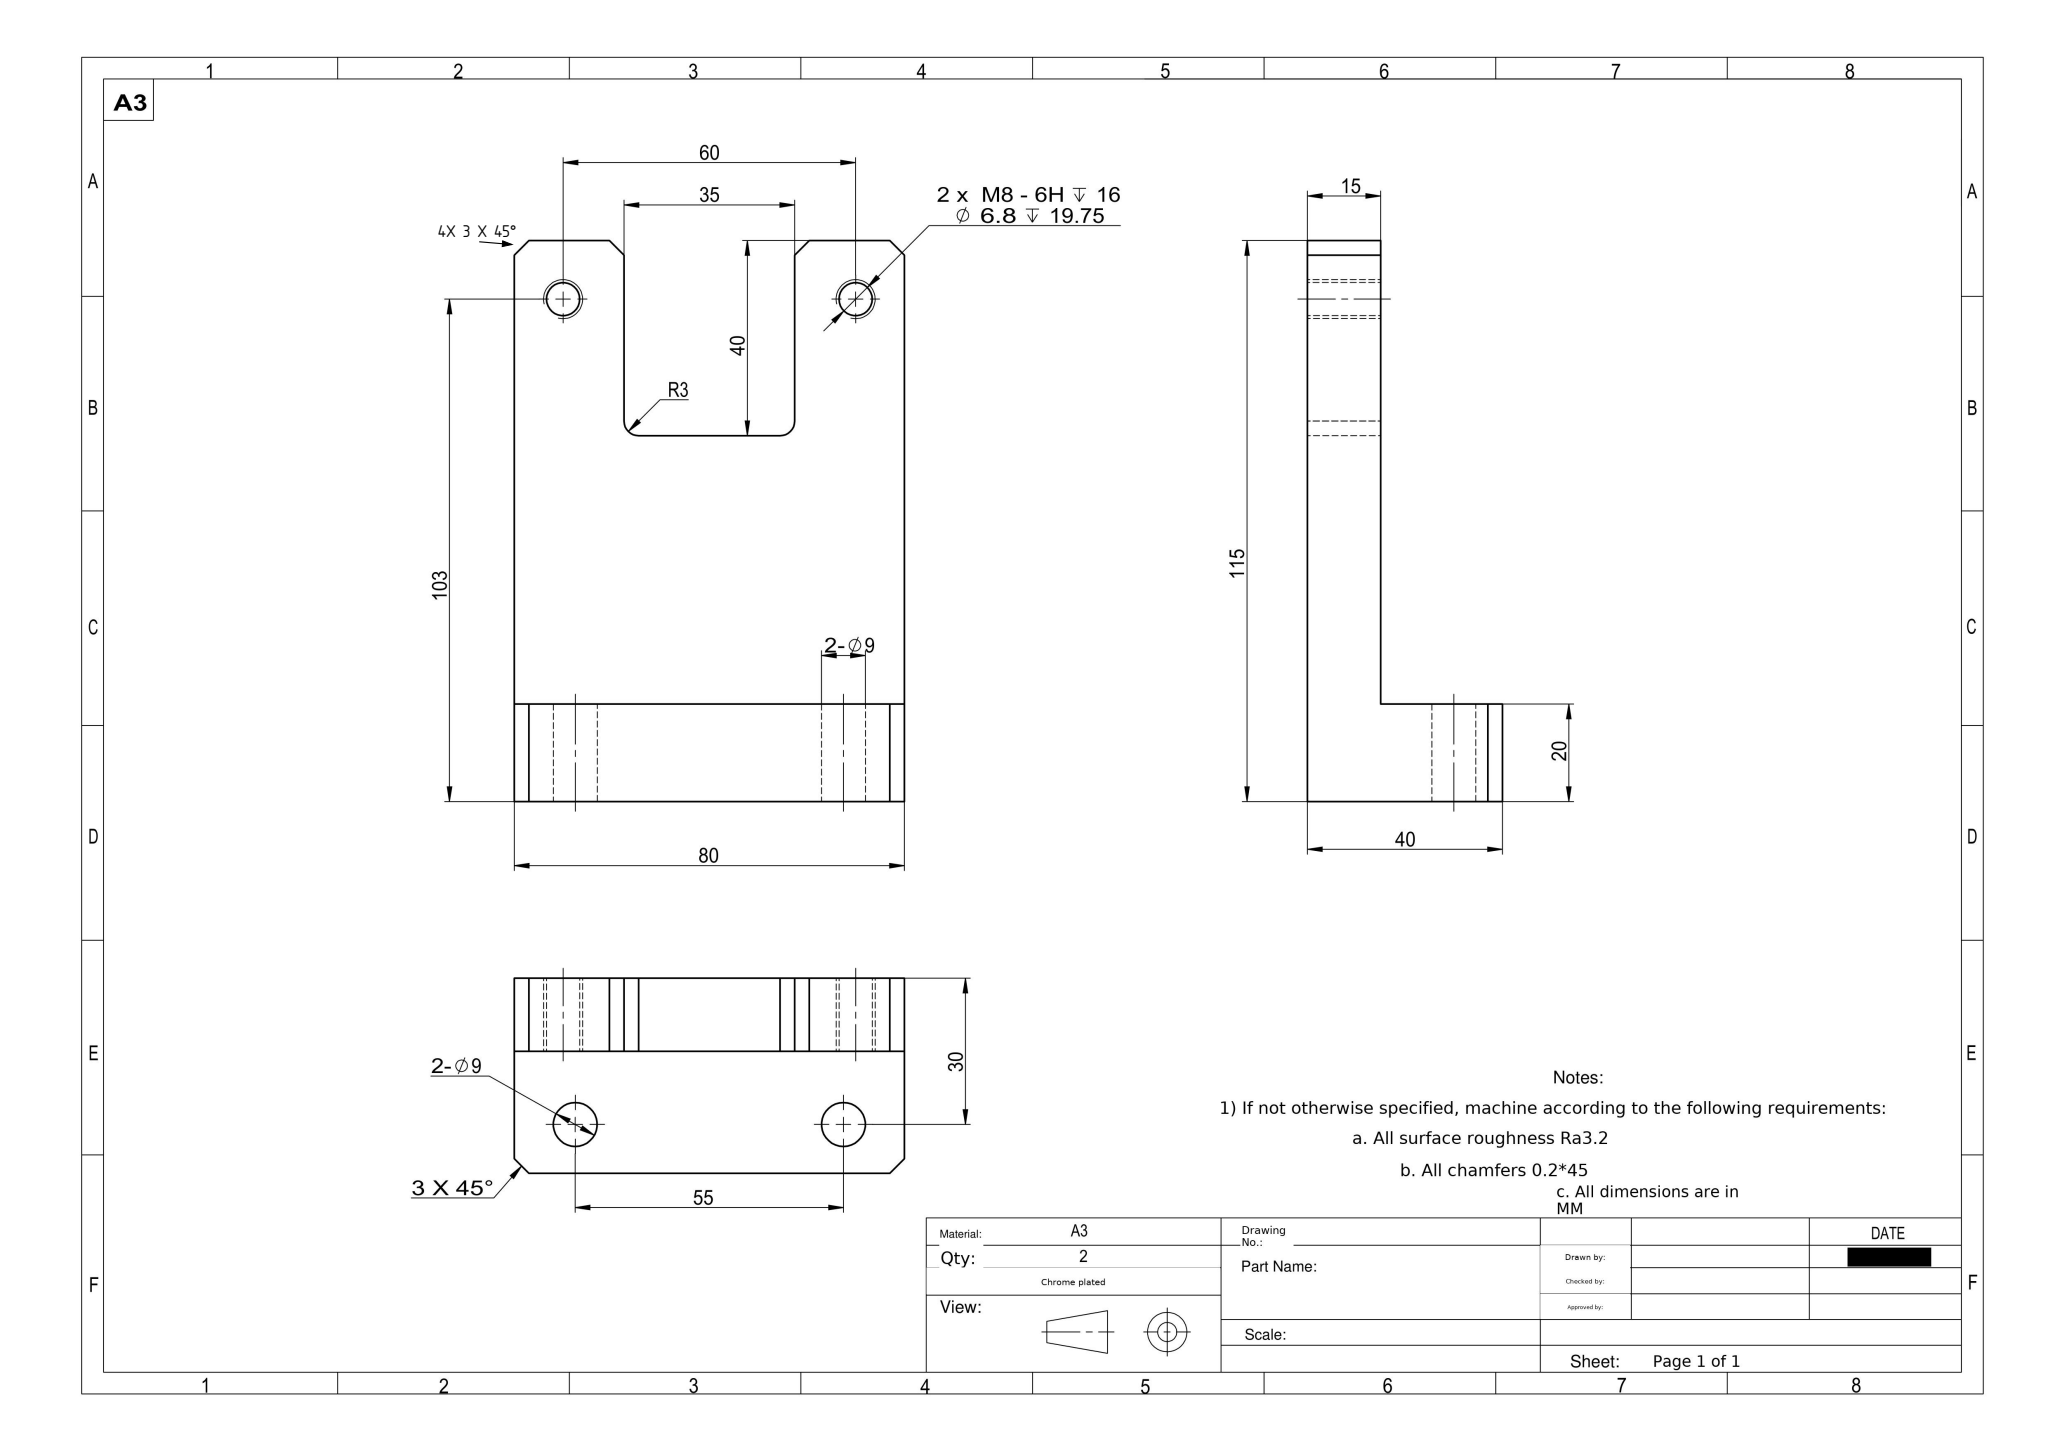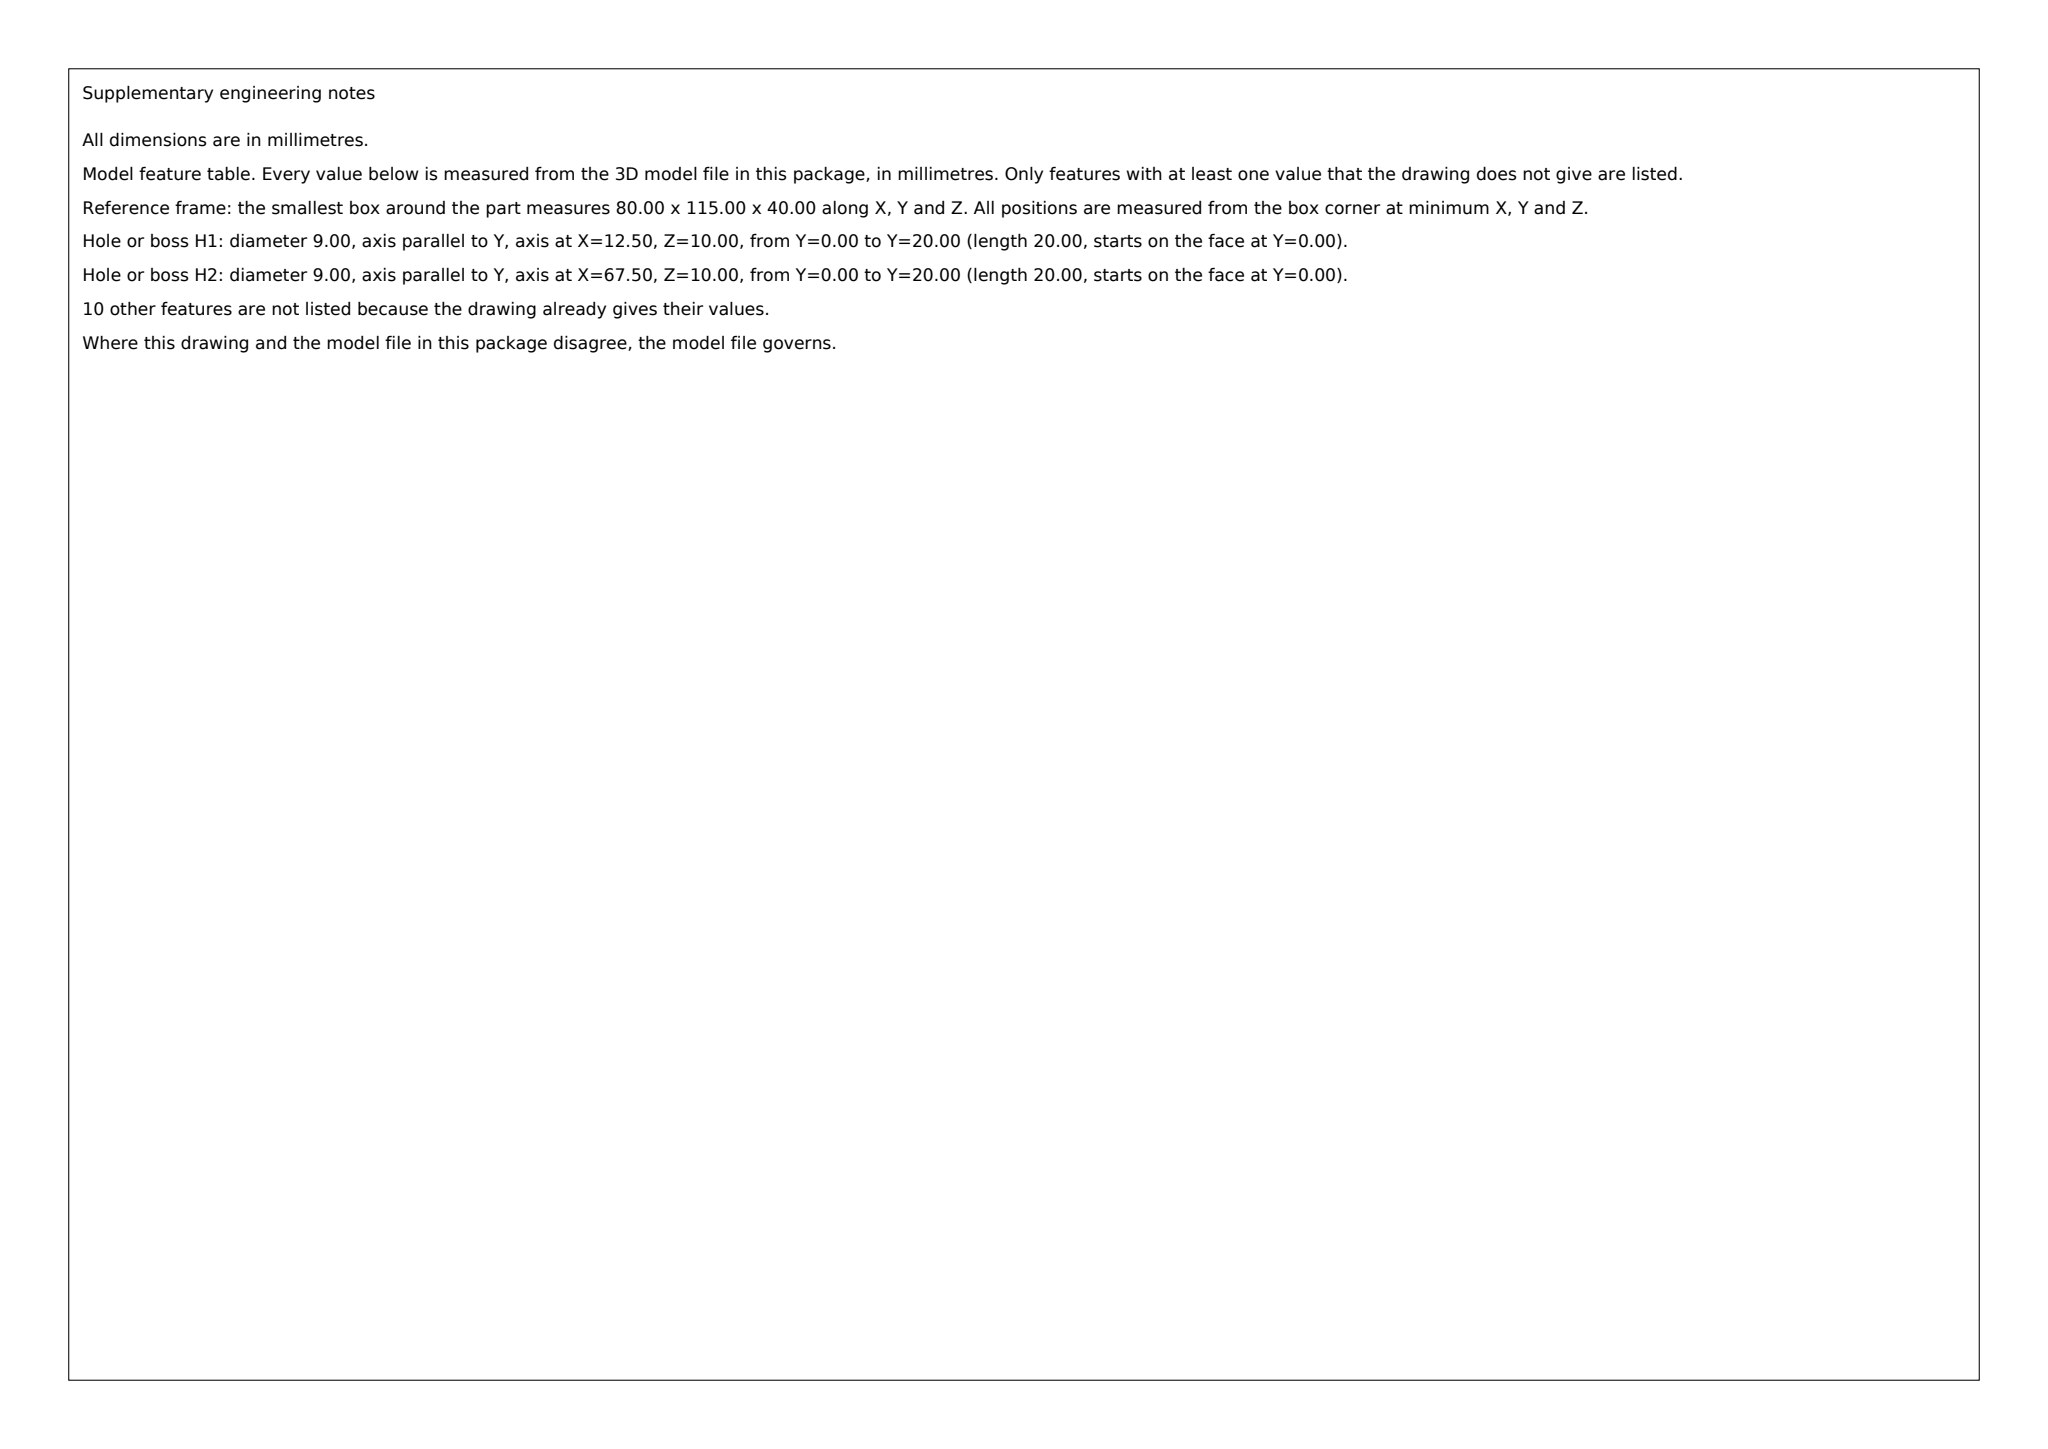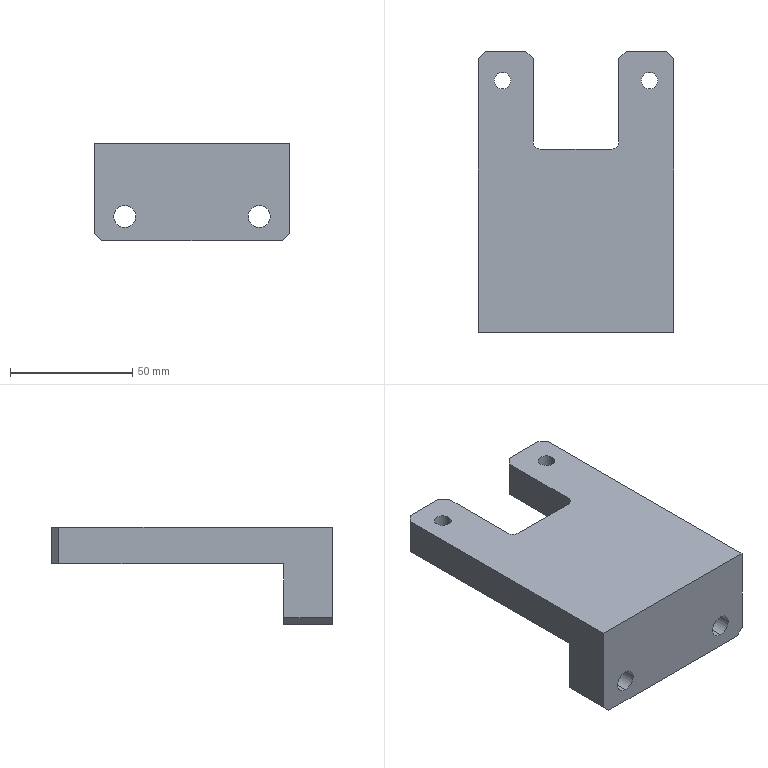Part | SolidWorks | mm | material A3 | 1 solid | 28 faces | box 80 x 115 x 40 mm | volume 152974 mm3 | plane 18 | cylinder 10 | commonest cylinder face diameters 6.8 x4 9 x4 6 x2
Drawing notes:
4X 3 X 45° CHAMFER ON TOP EDGE OF VERTICAL PLATE (15 THK), FULL THICKNESS; CHAMFER STARTS AT Y=112 FROM BOTTOM FACE, AT X=0, 19.5, 57.5 AND 77 FROM LEFT EDGE | from the solid: inclined_planes 4X angle_to_xyz_axes [45,45,90], bbox_from [0,112,25], [19.5,112,25], [57.5,112,25], [77,112,25], size [3,3,15]
build123d program:
from build123d import *

# Parameters (mm, degrees)
BOSS_EXTRUDE1_DEPTH          = 40
F_9_0_9_DIAMETER_HOLE1_D     = 9
F_9_0_9_DIAMETER_HOLE1_DEPTH = 27.5
F_9_0_9_DIAMETER_HOLE1_TIP   = 2.704
M8_TAPPED_HOLE1_D            = 6.8
M8_TAPPED_HOLE1_DEPTH        = 19.75
M8_TAPPED_HOLE1_TIP          = 2.043
SKETCH6_W                    = 35
SKETCH6_H                    = 40
CUT_EXTRUDE1_DEPTH           = 129.16
CHAMFER1_SIZE                = 3
FILLET1_R                    = 3


with BuildPart() as part:
    # Sketch1 → Boss-Extrude1 (new, symmetric)
    with BuildSketch(Plane(origin=(0, 0, 0), x_dir=(0, 0, -1), z_dir=(1, 0, 0))):
        Polygon((0, 0), (0, 115), (15, 115), (15, 20), (40, 20), (40, 0), align=None)
    extrude(amount=BOSS_EXTRUDE1_DEPTH, both=True)

    # 9.0 _9_ Diameter Hole1
    with Locations(Plane(origin=(0, 20, 0), x_dir=(1, 0, 0), z_dir=(0, 1, 0))):
        with Locations((27.5, 30), (-27.5, 30)):
            Hole(F_9_0_9_DIAMETER_HOLE1_D / 2, depth=F_9_0_9_DIAMETER_HOLE1_DEPTH)
            with Locations((0, 0, -(F_9_0_9_DIAMETER_HOLE1_DEPTH + F_9_0_9_DIAMETER_HOLE1_TIP / 2))):  # 118° drill point
                Cone(0, F_9_0_9_DIAMETER_HOLE1_D / 2, F_9_0_9_DIAMETER_HOLE1_TIP, mode=Mode.SUBTRACT)

    # M8 Tapped Hole1
    with Locations(Plane.XY):
        with Locations((30, 103), (-30, 103)):
            Hole(M8_TAPPED_HOLE1_D / 2, depth=M8_TAPPED_HOLE1_DEPTH)
            with Locations((0, 0, -(M8_TAPPED_HOLE1_DEPTH + M8_TAPPED_HOLE1_TIP / 2))):  # 118° drill point
                Cone(0, M8_TAPPED_HOLE1_D / 2, M8_TAPPED_HOLE1_TIP, mode=Mode.SUBTRACT)

    # Sketch6 → Cut-Extrude1 (cut, through all)
    with BuildSketch(Plane.XY):
        with Locations((0, 95)):
            Rectangle(SKETCH6_W, SKETCH6_H)
    extrude(amount=-CUT_EXTRUDE1_DEPTH, mode=Mode.SUBTRACT)

    # Chamfer1
    chamfer1_edges = [part.edges().sort_by_distance(p)[0] for p in [
        (40, 115, -7.5),
        (-17.5, 115, -7.5),
        (17.5, 115, -7.5),
        (-40, 115, -7.5),
        (40, 10, -40),
        (-40, 10, -40),
    ]]
    chamfer(chamfer1_edges, length=CHAMFER1_SIZE)

    # Fillet1
    fillet1_edges = [part.edges().sort_by_distance(p)[0] for p in [
        (-17.5, 75, -7.5),
        (17.5, 75, -7.5),
    ]]
    fillet(fillet1_edges, radius=FILLET1_R)


solid = part.part